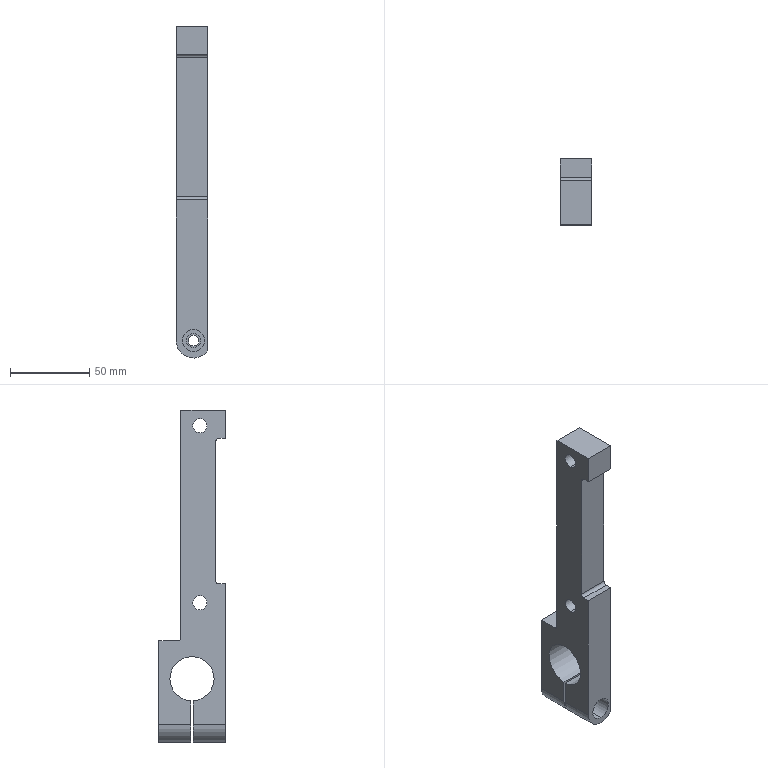Component | SolidWorks | 21MicrometerFrame-1 | 1 solid | 38 faces | box 20 x 42 x 210 mm | volume 102593 mm3 | cylinder 20 | plane 16 | cone 2 | commonest cylinder face diameters 14 x6 9 x6 4 x3 6.8 x2 22 x2 28 x1
build123d program:
from build123d import *

# Parameters (mm, degrees)
SKETCH1_W                   = 210
SKETCH1_H                   = 42
BOSS_EXTRUDE1_DEPTH         = 20
CUT_EXTRUDE1_DEPTH          = 22
CUT_EXTRUDE3_DEPTH          = 99
SKETCH4_W                   = 43.331
SKETCH4_H                   = 1.5
CUT_EXTRUDE4_DEPTH          = 99
SKETCH5_R                   = 7
CUT_EXTRUDE5_DEPTH          = 10
SKETCH6_R                   = 4.5
CUT_EXTRUDE6_DEPTH          = 11
M8_TAPPED_HOLE1_D           = 6.8
M8_TAPPED_HOLE1_DEPTH       = 21
M8_TAPPED_HOLE1_CSINK_D     = 8.05
M8_TAPPED_HOLE1_CSINK_ANGLE = 90
M8_TAPPED_HOLE1_TIP         = 2.043
HOLE1_D                     = 9
HOLE1_DEPTH                 = 100
HOLE1_CBORE_D               = 14
HOLE1_CBORE_DEPTH           = 10


with BuildPart() as part:
    # Sketch1 → Boss-Extrude1 (new body)
    with BuildSketch(Plane.XY):
        with Locations((-105, -21)):
            Rectangle(SKETCH1_W, SKETCH1_H)
    extrude(amount=BOSS_EXTRUDE1_DEPTH)

    # Sketch2 → Cut-Extrude1 (cut)
    with BuildSketch(Plane.XY.offset(20)):
        with BuildLine():
            Line((-210, 0), (-64, 0))
            Line((-64, 0), (-64, -12))
            ThreePointArc((-64, -12), (-64.586, -13.414), (-66, -14))
            Line((-66, -14), (-210, -14))
            Line((-210, -14), (-210, 0))
        make_face()
        with BuildLine():
            Line((-192, -42), (-100, -42))
            Line((-100, -42), (-100, -38))
            ThreePointArc((-100, -38), (-100.586, -36.586), (-102, -36))
            Line((-102, -36), (-190, -36))
            ThreePointArc((-190, -36), (-191.414, -36.586), (-192, -38))
            Line((-192, -38), (-192, -42))
        make_face()
    extrude(amount=-CUT_EXTRUDE1_DEPTH, mode=Mode.SUBTRACT)

    # Sketch3 → Cut-Extrude3 (cut)
    with BuildSketch(Plane(origin=(0, 0, 0), x_dir=(1, 0, 0), z_dir=(0, 1, 0))):
        with BuildLine():
            Line((0, 0), (-11, 0))
            ThreePointArc((-11, 0), (-3.222, -3.222), (0, -11))
            Line((0, -11), (0, 0))
        make_face()
        with BuildLine():
            Line((0, -20), (0, -11))
            ThreePointArc((0, -11), (-1.239, -16.071), (-4.675, -20))
            Line((-4.675, -20), (0, -20))
        make_face()
    extrude(amount=-CUT_EXTRUDE3_DEPTH, mode=Mode.SUBTRACT)

    # Sketch4 → Cut-Extrude4 (cut)
    with BuildSketch(Plane.XY.offset(20)):
        with BuildLine():
            Line((-38.656, -21.75), (-38.656, -20.25))
            Line((-38.656, -20.25), (-26.02, -20.25))
            ThreePointArc((-26.02, -20.25), (-54, -21), (-26.02, -21.75))
            Line((-26.02, -21.75), (-38.656, -21.75))
        make_face()
        with BuildLine():
            Line((-26.02, -20.25), (-38.656, -20.25))
            Line((-38.656, -20.25), (-38.656, -21.75))
            Line((-38.656, -21.75), (-26.02, -21.75))
            ThreePointArc((-26.02, -21.75), (-26.005, -21.375), (-26, -21))
            ThreePointArc((-26, -21), (-26.005, -20.625), (-26.02, -20.25))
        make_face()
        with BuildLine():
            Line((-4.675, -20.25), (-26.02, -20.25))
            ThreePointArc((-26.02, -20.25), (-26.005, -20.625), (-26, -21))
            ThreePointArc((-26, -21), (-26.005, -21.375), (-26.02, -21.75))
            Line((-26.02, -21.75), (-4.675, -21.75))
            Line((-4.675, -21.75), (-4.675, -20.25))
        make_face()
        with BuildLine():
            Line((-38.656, -21.75), (-38.656, -20.25))
            Line((-38.656, -20.25), (-26.02, -20.25))
            ThreePointArc((-26.02, -20.25), (-54, -21), (-26.02, -21.75))
            Line((-26.02, -21.75), (-38.656, -21.75))
        make_face()
        with BuildLine():
            Line((-26.02, -20.25), (-38.656, -20.25))
            Line((-38.656, -20.25), (-38.656, -21.75))
            Line((-38.656, -21.75), (-26.02, -21.75))
            ThreePointArc((-26.02, -21.75), (-26.005, -21.375), (-26, -21))
            ThreePointArc((-26, -21), (-26.005, -20.625), (-26.02, -20.25))
        make_face()
        with Locations((16.99, -21)):
            Rectangle(SKETCH4_W, SKETCH4_H)
    extrude(amount=-CUT_EXTRUDE4_DEPTH, mode=Mode.SUBTRACT)

    # Sketch5 → Cut-Extrude5 (cut)
    with BuildSketch(Plane.XZ.offset(42)):
        with Locations((-11, 11)):
            Circle(SKETCH5_R)
    extrude(amount=-CUT_EXTRUDE5_DEPTH, mode=Mode.SUBTRACT)

    # Sketch6 → Cut-Extrude6 (cut)
    with BuildSketch(Plane.XZ.offset(32)):
        with Locations((-11, 11)):
            Circle(SKETCH6_R)
    extrude(amount=-CUT_EXTRUDE6_DEPTH, mode=Mode.SUBTRACT)

    # M8 Tapped Hole1
    with Locations(Plane(origin=(0, 0, 0), x_dir=(1, 0, 0), z_dir=(0, 1, 0))):
        with Locations((-11, -11)):
            CounterSinkHole(M8_TAPPED_HOLE1_D / 2, M8_TAPPED_HOLE1_CSINK_D / 2, depth=M8_TAPPED_HOLE1_DEPTH, counter_sink_angle=M8_TAPPED_HOLE1_CSINK_ANGLE)
            with Locations((0, 0, -(M8_TAPPED_HOLE1_DEPTH + M8_TAPPED_HOLE1_TIP / 2))):  # 118° drill point
                Cone(0, M8_TAPPED_HOLE1_D / 2, M8_TAPPED_HOLE1_TIP, mode=Mode.SUBTRACT)

    # Hole1
    with Locations(Plane.XY.offset(20)):
        with Locations((-88, -26), (-200, -26)):
            CounterBoreHole(HOLE1_D / 2, HOLE1_CBORE_D / 2, HOLE1_CBORE_DEPTH, depth=HOLE1_DEPTH)


solid = part.part

# Placed as in the assembly
solid = solid.moved(Location((145.283, 124, -139), (0, 90, 0)))